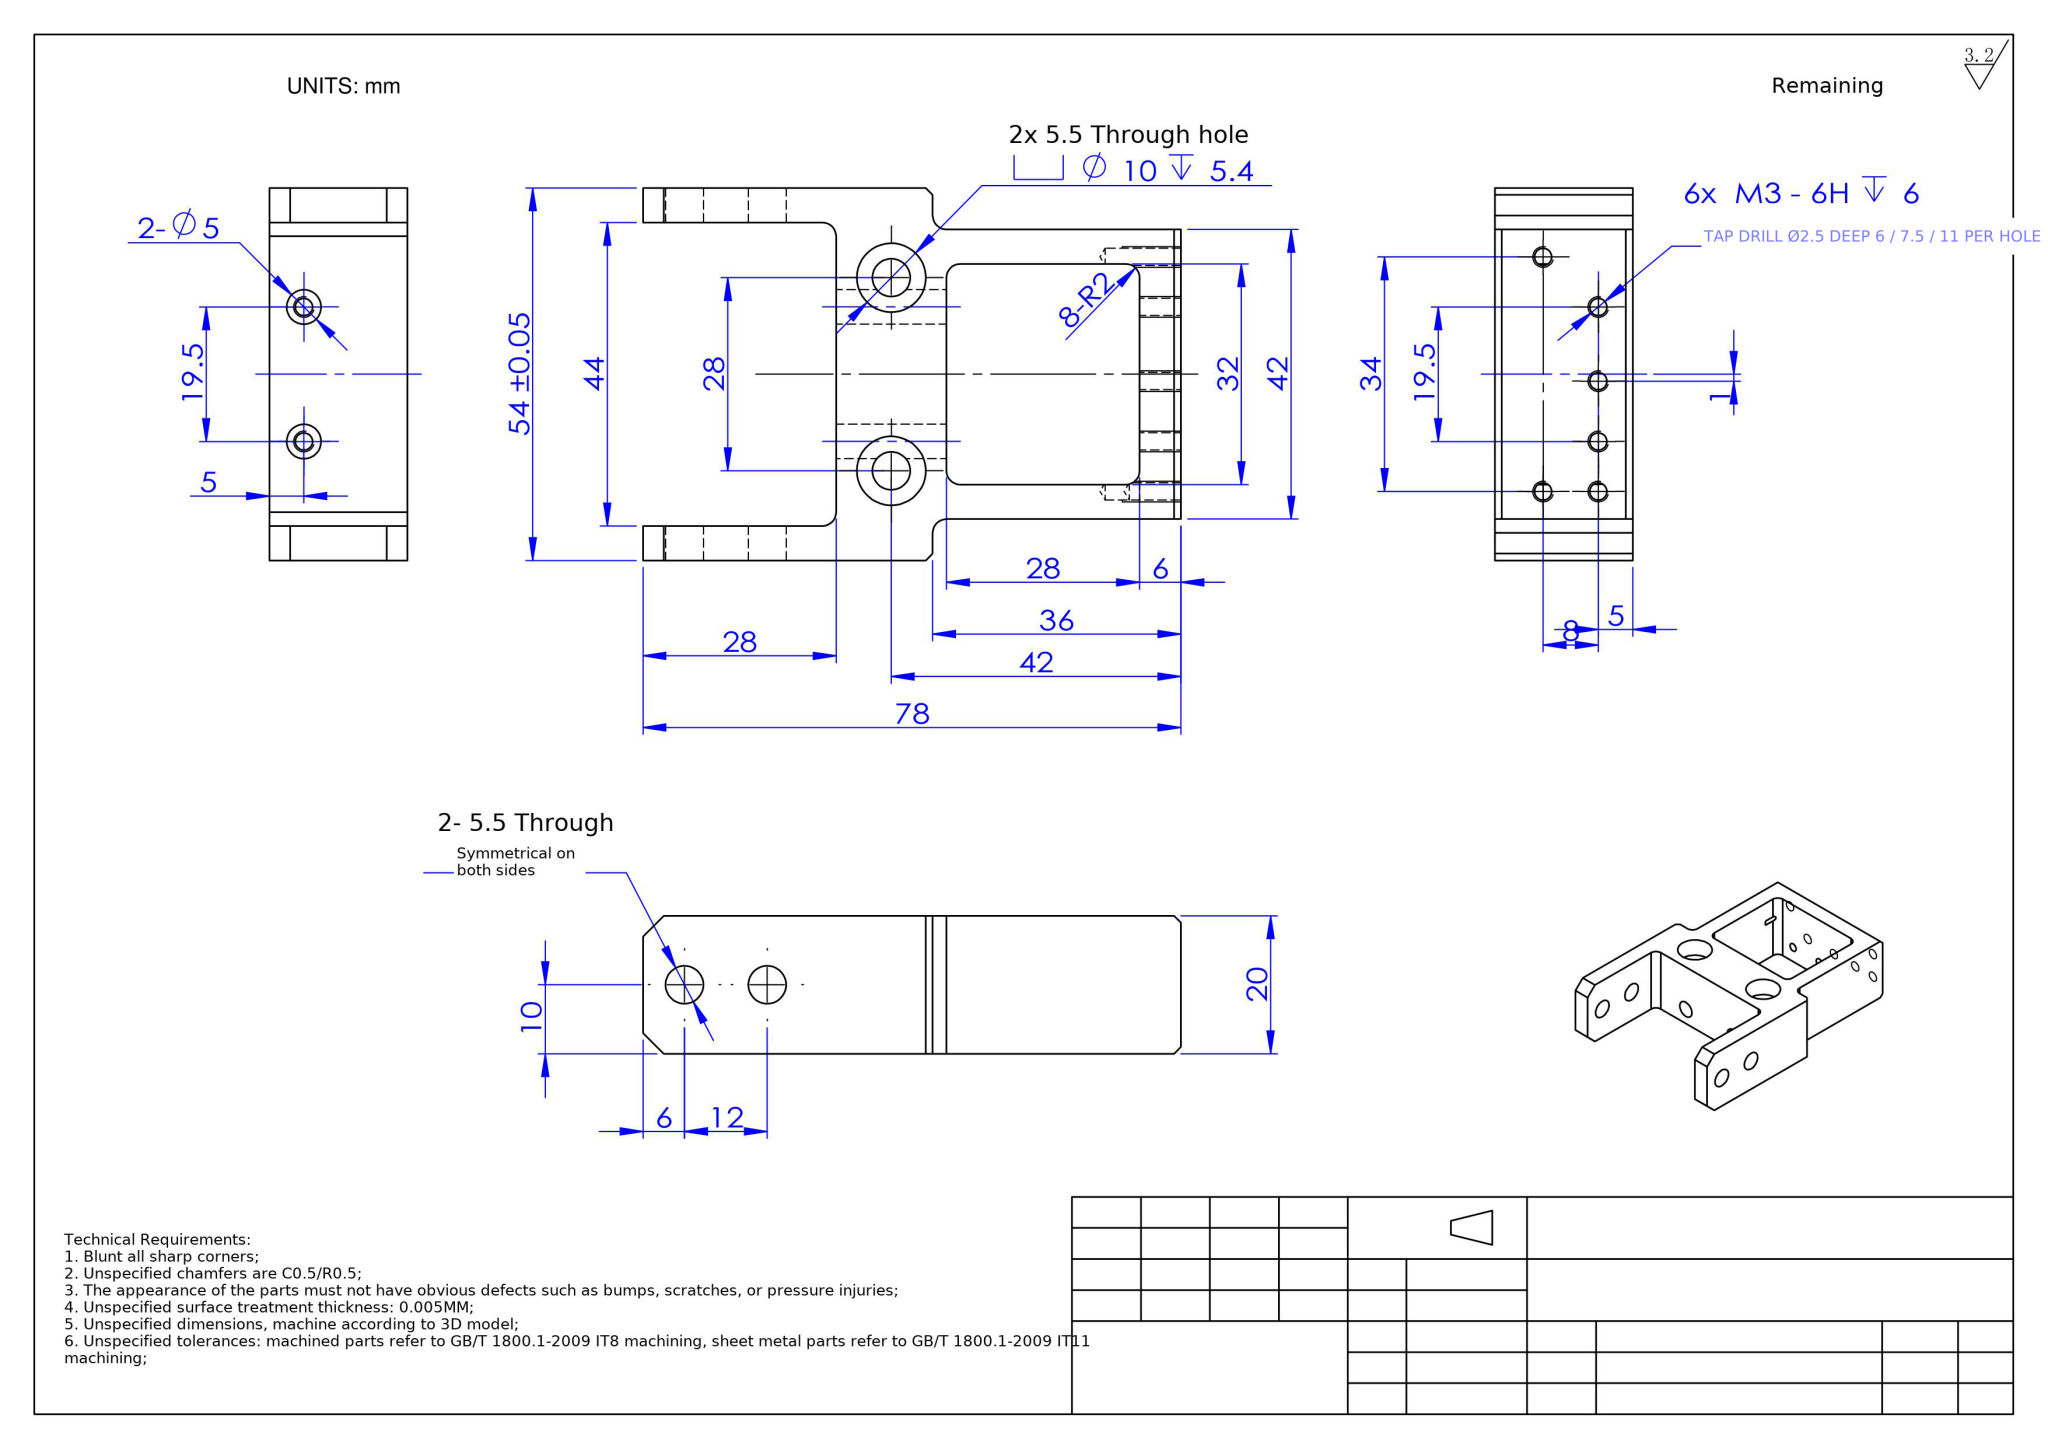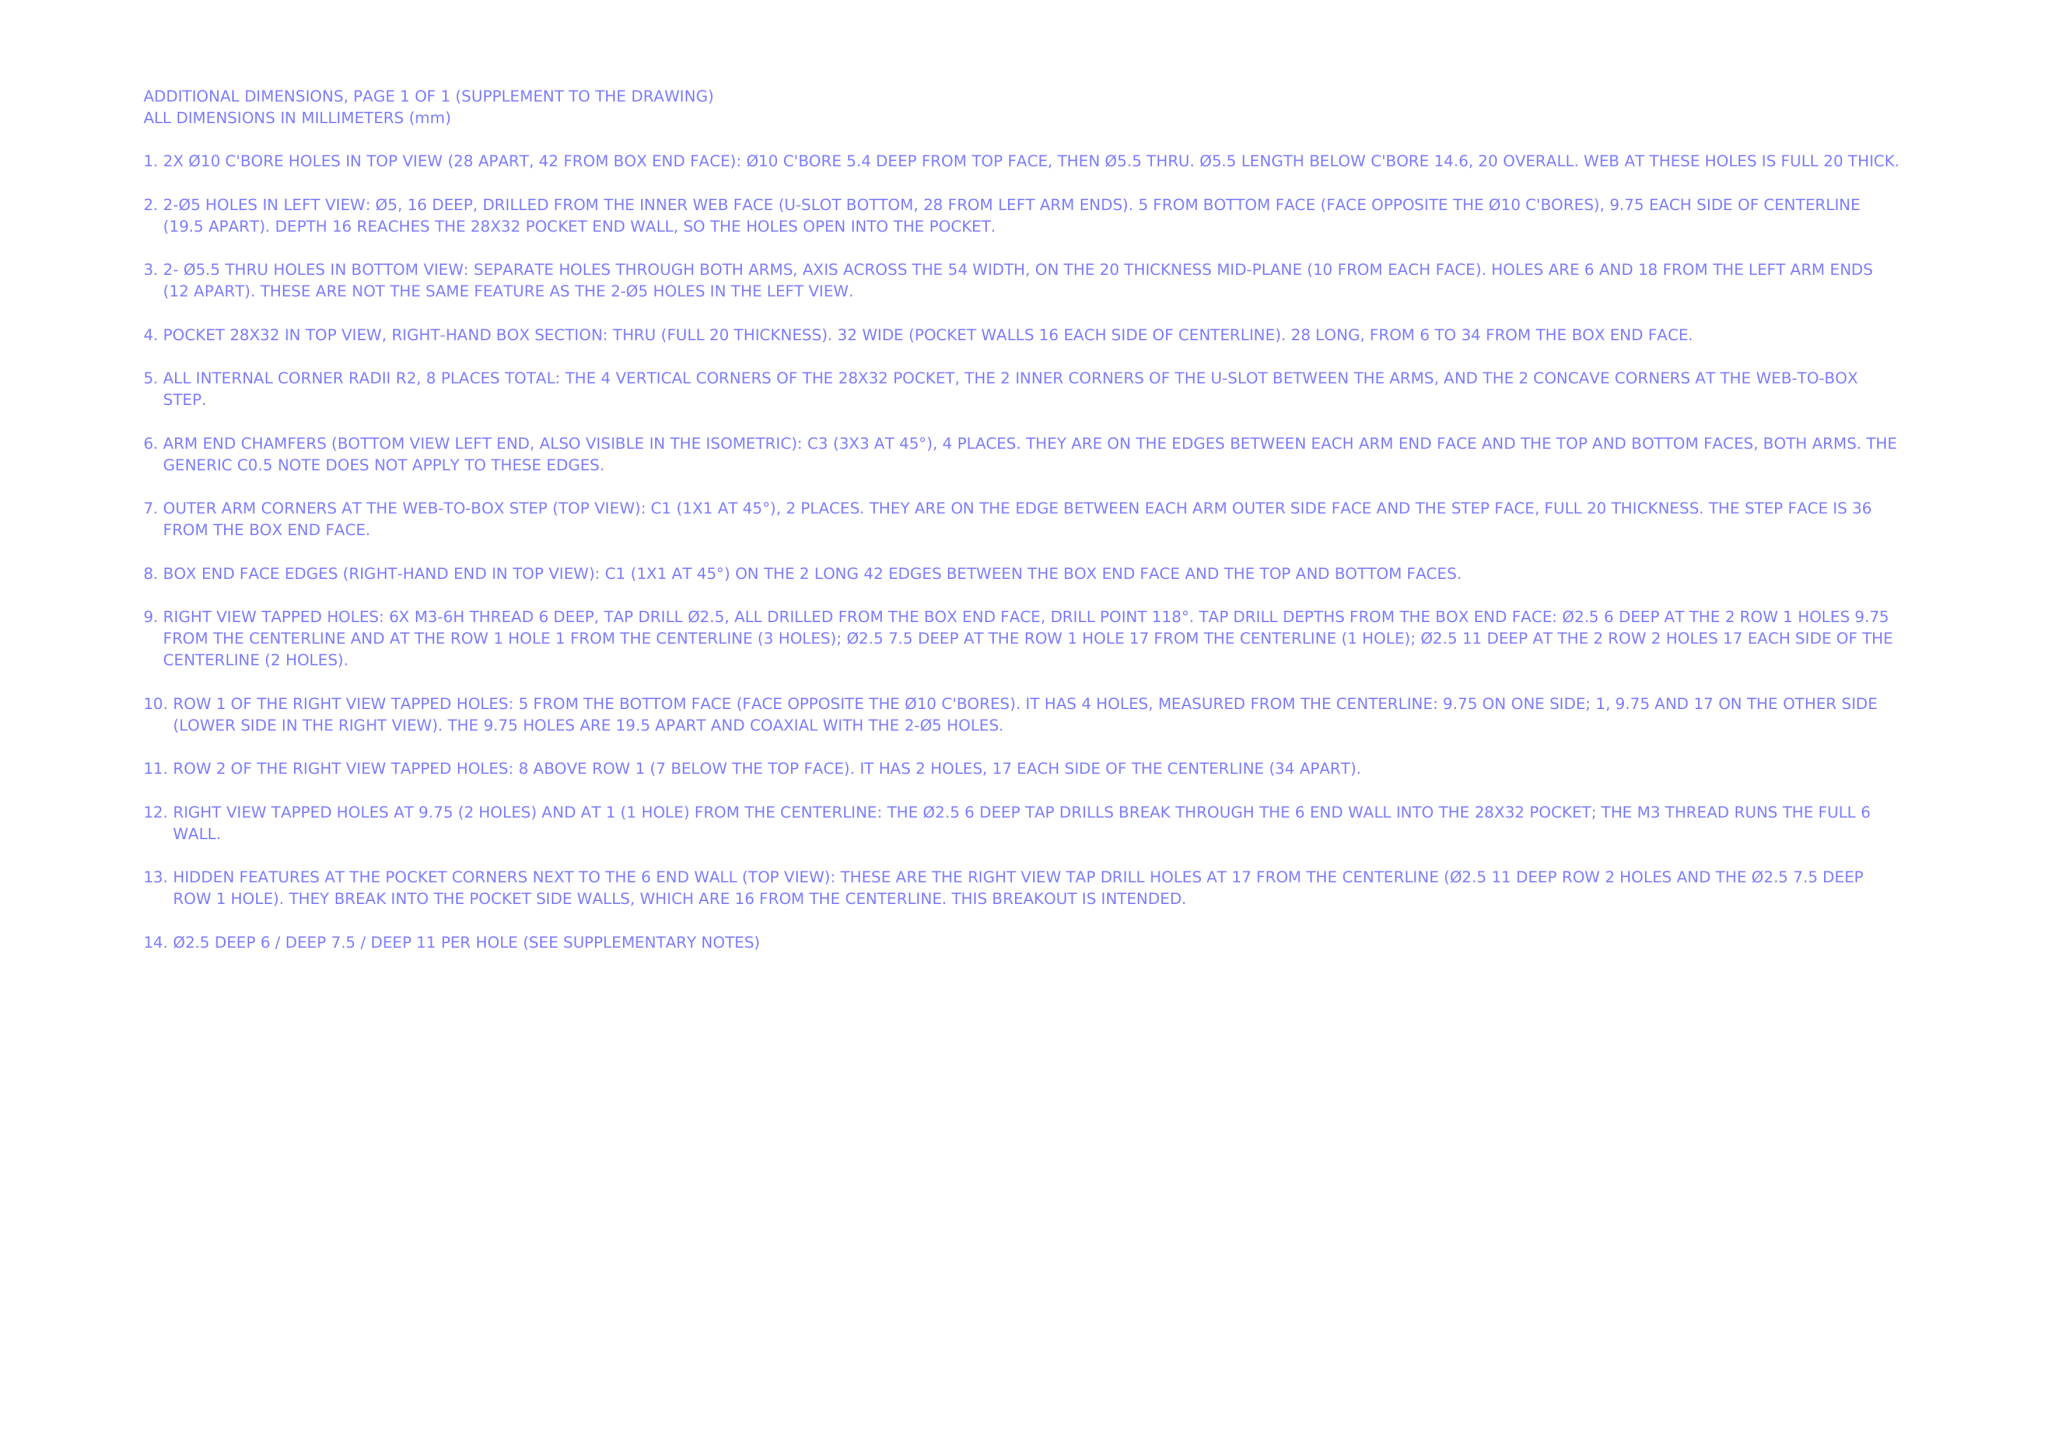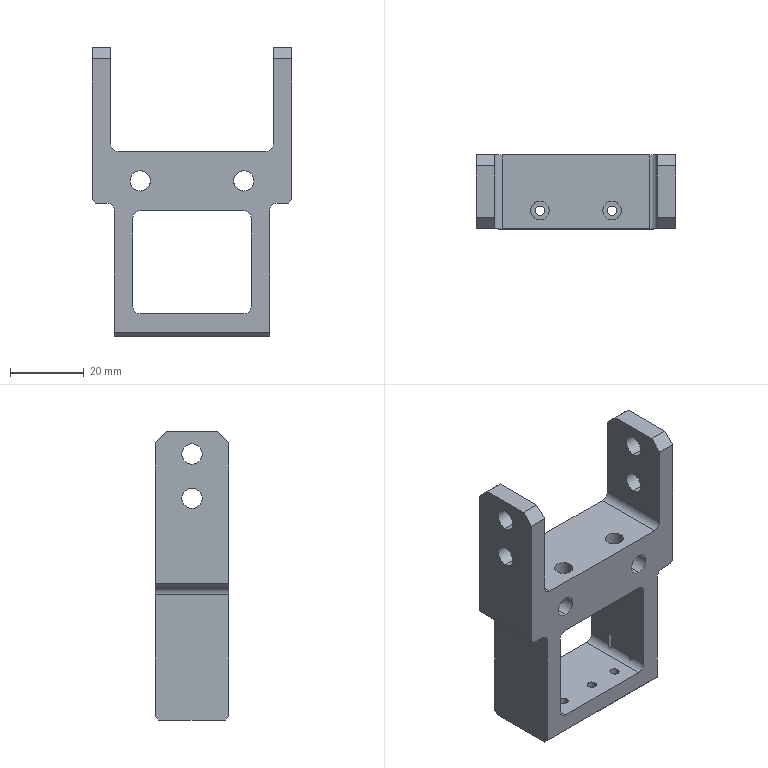Part | NX | mm | 1 solid | 74 faces | box 54 x 20 x 78 mm | volume 30160 mm3 | cylinder 40 | plane 28 | cone 6 | commonest cylinder face diameters 5.5 x12 2.5 x12 4 x8 5 x4 10 x4